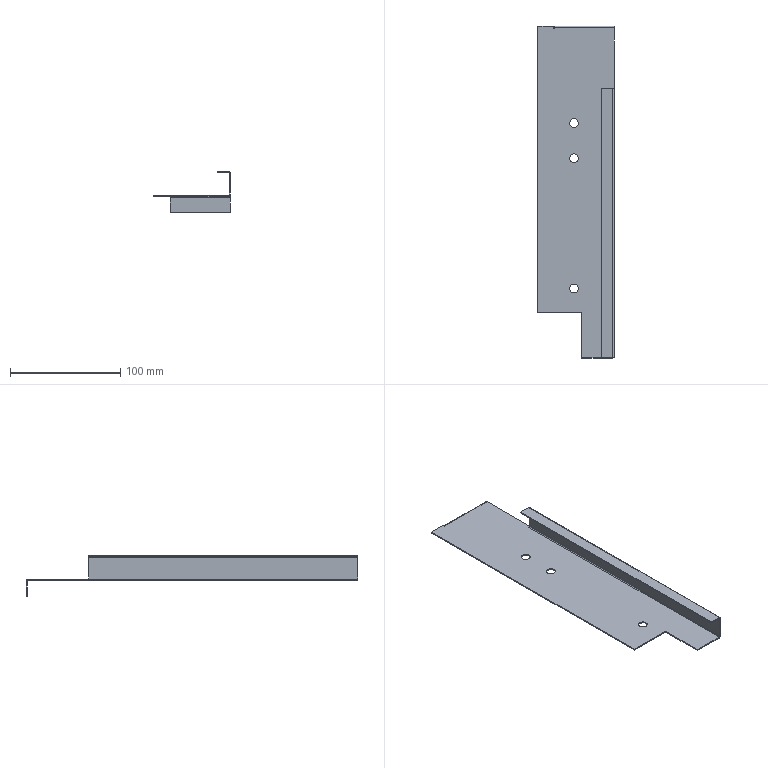Component | SolidWorks | CCQ-1.1-6SideUpperPlate4-1 | 1 solid | 46 faces | volume 27654 mm3 | plane 34 | cylinder 12 | commonest cylinder face diameters 8 x6 3.473 x3 1.473 x3 | material 304